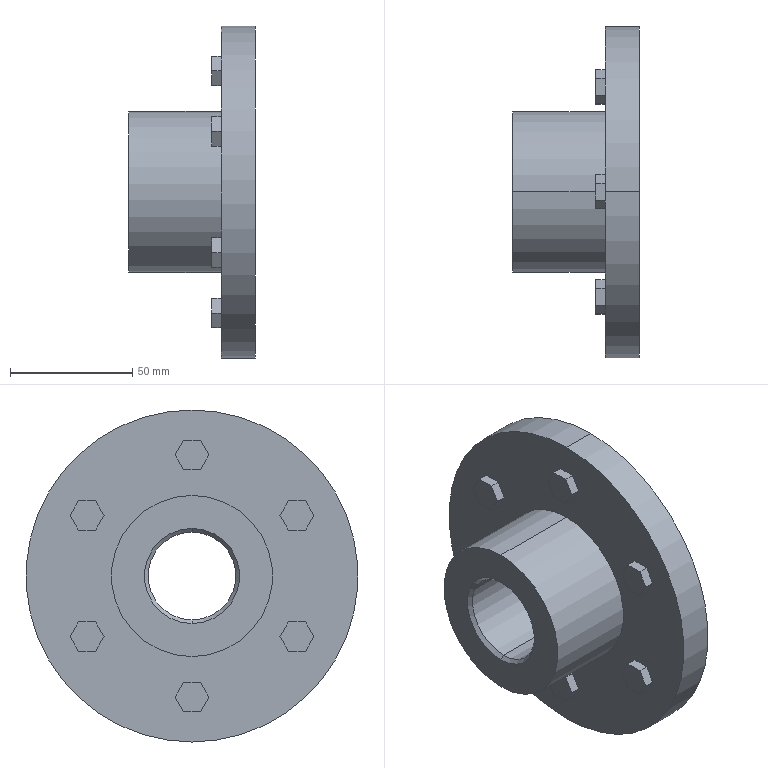Component | SolidWorks | Coupling-1 | 1 solid | 53 faces | box 52 x 136 x 136 mm | volume 283332 mm3 | plane 45 | cylinder 6 | cone 2 | commonest cylinder face diameters 136 x2 36 x2 66 x2
build123d program:
from build123d import *

# Parameters (mm, degrees)
SKETCH1_R           = 33
SKETCH1_R_2         = 18
BOSS_EXTRUDE1_DEPTH = 38
SKETCH2_R           = 68
SKETCH2_R_2         = 18
BOSS_EXTRUDE2_DEPTH = 14
BOSS_EXTRUDE3_DEPTH = 4
CHAMFER1_SIZE       = 1.5


with BuildPart() as part:
    # Sketch1 → Boss-Extrude1 (new body)
    with BuildSketch(Plane(origin=(0, 0, 0), x_dir=(0, 0, -1), z_dir=(1, 0, 0))):
        Circle(SKETCH1_R)
        Circle(SKETCH1_R_2, mode=Mode.SUBTRACT)
    extrude(amount=BOSS_EXTRUDE1_DEPTH)

    # Sketch2 → Boss-Extrude2 (add)
    with BuildSketch(Plane(origin=(38, 0, 0), x_dir=(0, 0, -1), z_dir=(1, 0, 0))):
        Circle(SKETCH2_R)
        Circle(SKETCH2_R_2, mode=Mode.SUBTRACT)
    extrude(amount=BOSS_EXTRUDE2_DEPTH)

    # Sketch3 → Boss-Extrude3 (add)
    with BuildSketch(Plane.ZY.offset(-38)):
        Polygon((18.799, -46.463), (24.819, -49.939), (30.839, -46.463), (30.839, -39.512), (24.819, -36.036), (18.799, -39.512), align=None)
        Polygon((49.638, -6.952), (55.658, -3.476), (55.658, 3.476), (49.638, 6.952), (43.617, 3.476), (43.617, -3.476), align=None)
        Polygon((-30.839, -39.512), (-30.839, -46.463), (-24.819, -49.939), (-18.799, -46.463), (-18.799, -39.512), (-24.819, -36.036), align=None)
        Polygon((-49.638, 6.952), (-55.658, 3.476), (-55.658, -3.476), (-49.638, -6.952), (-43.617, -3.476), (-43.617, 3.476), align=None)
        Polygon((-18.799, 46.463), (-24.819, 49.939), (-30.839, 46.463), (-30.839, 39.512), (-24.819, 36.036), (-18.799, 39.512), align=None)
        Polygon((30.839, 39.512), (30.839, 46.463), (24.819, 49.939), (18.799, 46.463), (18.799, 39.512), (24.819, 36.036), align=None)
    extrude(amount=BOSS_EXTRUDE3_DEPTH)

    # Chamfer1
    chamfer1_edges = [part.edges().sort_by_distance(p)[0] for p in [
        (0, 0, 18),
    ]]
    chamfer(chamfer1_edges, length=CHAMFER1_SIZE)


solid = part.part

# Placed as in the assembly
solid = solid.moved(Location((250.528, 15.31, -110), (0, 0, 0)))